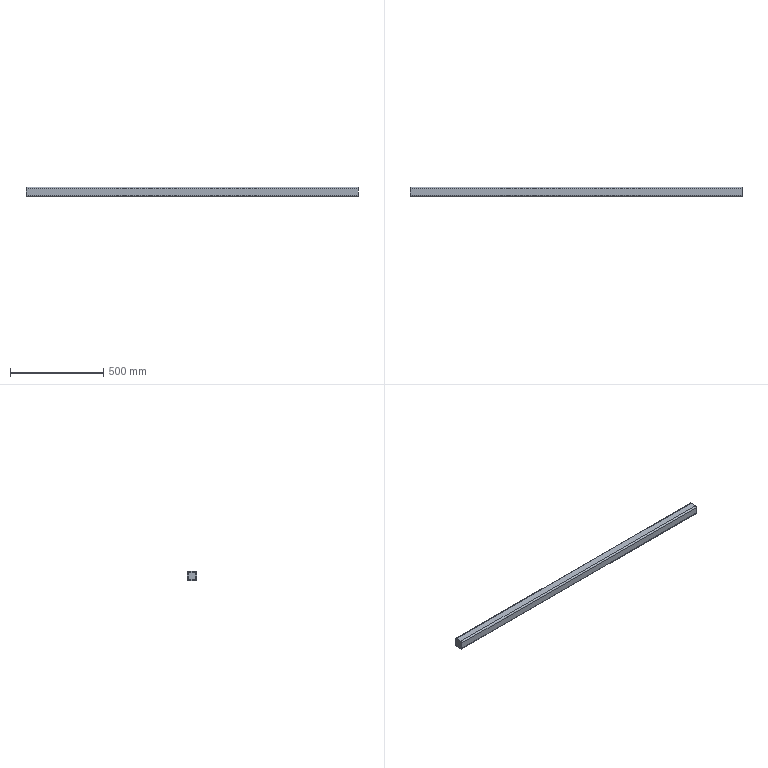Component | SolidWorks | AX00-100.1.1-1_AXFrame_A.1.1-1_AX50x50-2_square tube.1.1-3 | 1 solid | 20 faces | box 1780 x 50 x 50 mm | volume 1533885 mm3 | plane 12 | cylinder 8 | commonest cylinder face diameters 16 x4 6 x4 | material AISI 1035 Steel (SS)
build123d program:
from build123d import *

# Parameters (mm, degrees)
SKETCH1_W           = 50
SKETCH1_H           = 50
BOSS_EXTRUDE1_DEPTH = 890
FILLET3_R           = 8
SHELL1_T            = 5


with BuildPart() as part:
    # Sketch1 → Boss-Extrude1 (new, symmetric)
    with BuildSketch(Plane.XY):
        Rectangle(SKETCH1_W, SKETCH1_H)
    extrude(amount=BOSS_EXTRUDE1_DEPTH, both=True)

    # Fillet3
    fillet3_edges = [part.edges().sort_by_distance(p)[0] for p in [
        (25, -25, 0),
        (-25, -25, 0),
        (-25, 25, 0),
        (25, 25, 0),
    ]]
    fillet(fillet3_edges, radius=FILLET3_R)

    # Shell1 (no face opened: a closed hollow body)
    add(offset(amount=-SHELL1_T, mode=Mode.PRIVATE), mode=Mode.SUBTRACT)


solid = part.part

# Placed as in the assembly
solid = solid.moved(Location((228.631, -361.636, -197.5), (0, 90, 0)))